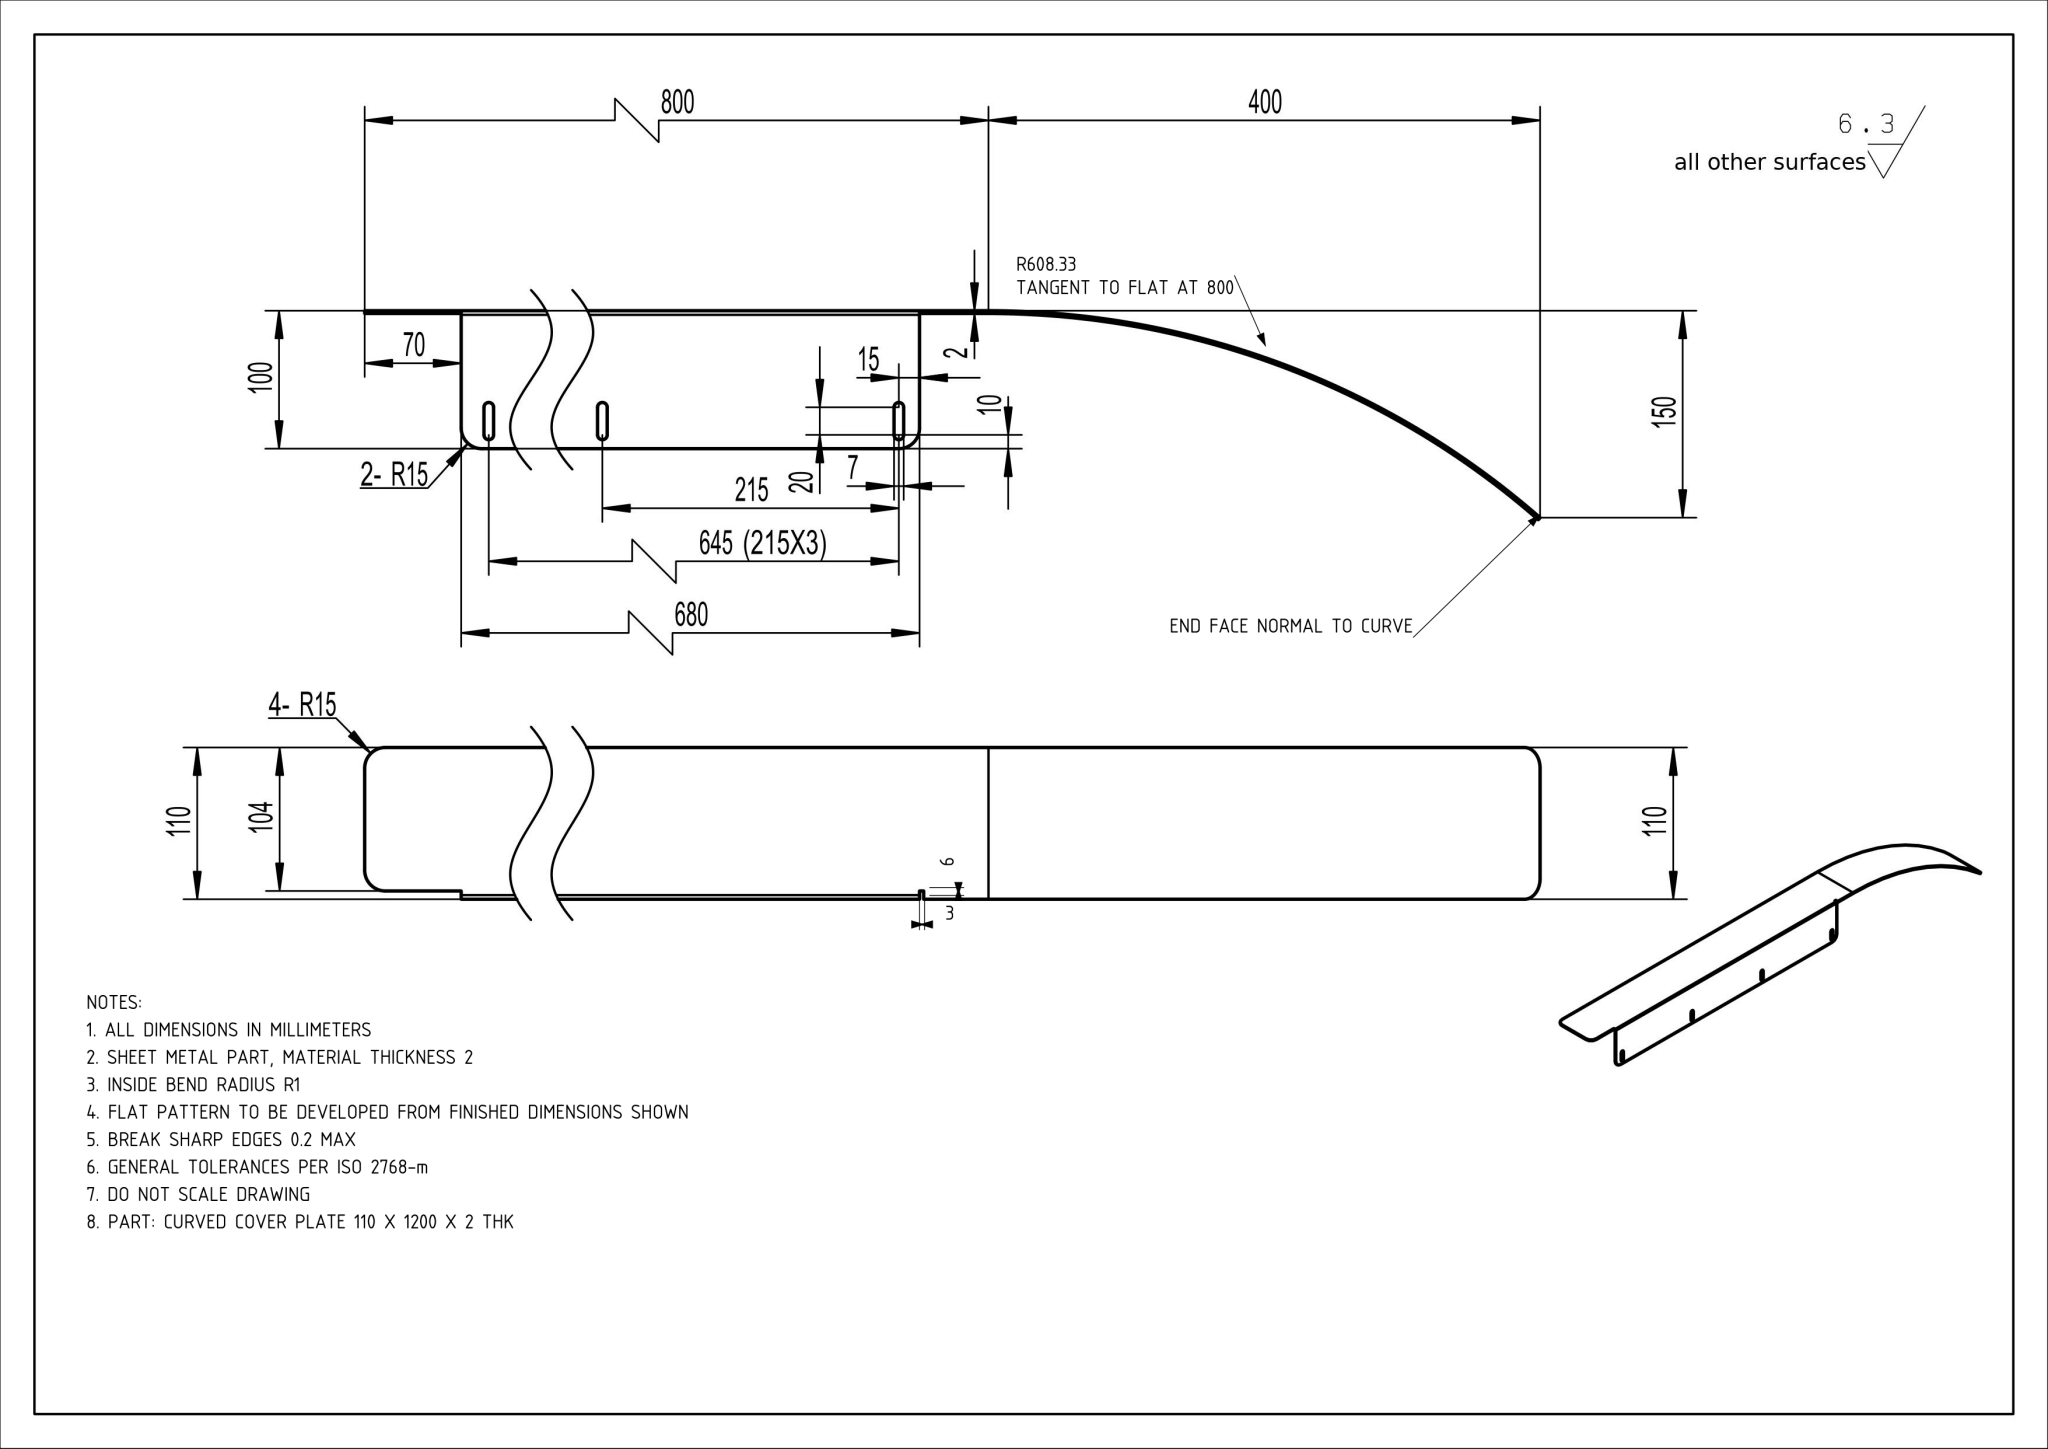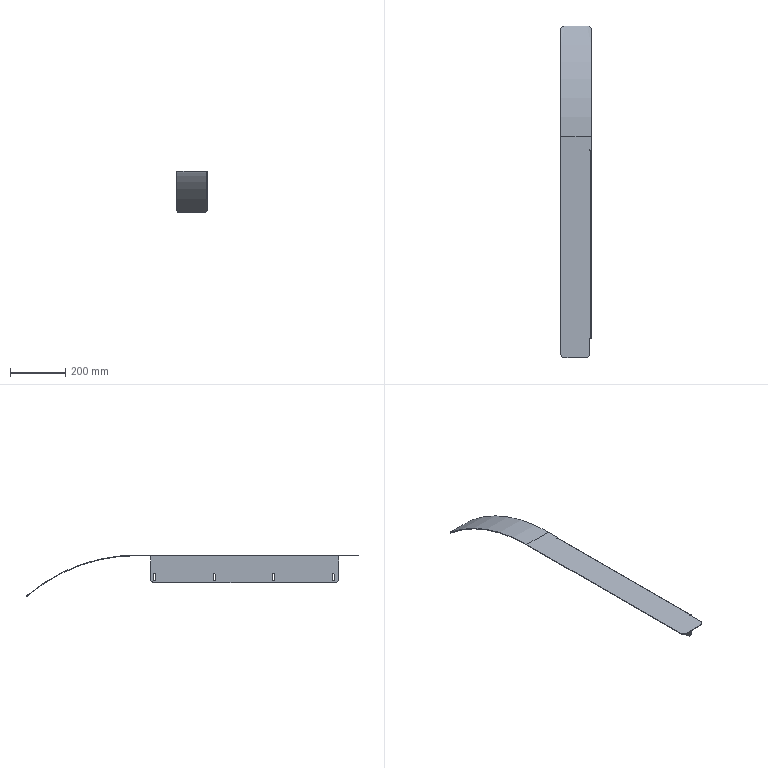Part | NX | mm | 1 solid | 40 faces | box 110 x 1200 x 151.51 mm | volume 401101 mm3 | plane 22 | cylinder 18 | commonest cylinder face diameters 7 x8 30 x6 1216.667 x1 1212.667 x1 2 x1 6 x1